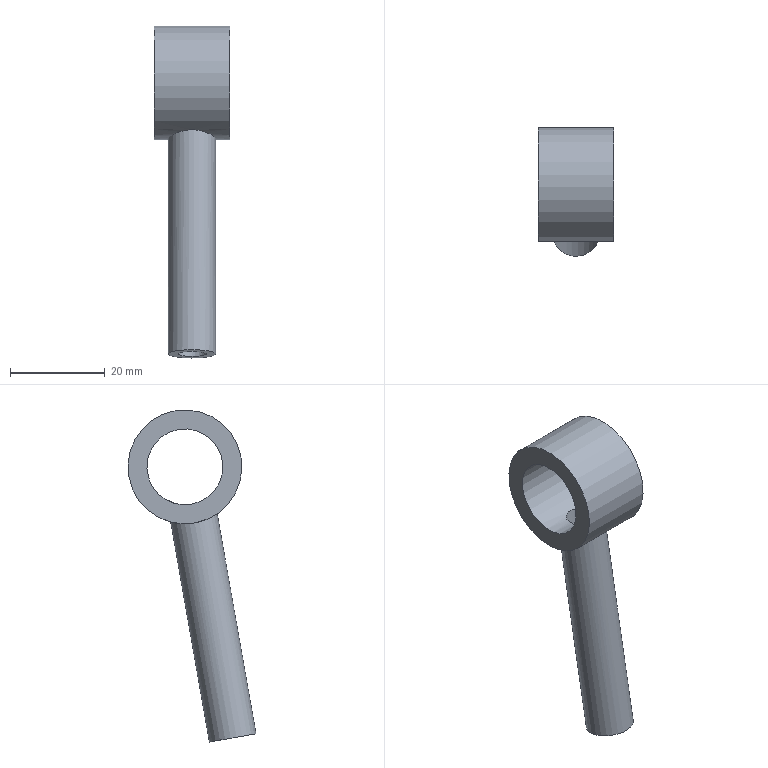Component | NX | SWING_ROD_2 | 1 solid | 7 faces | volume 6237 mm3 | cylinder 4 | plane 3 | commonest cylinder face diameters 24 x1 16 x1 10 x1 6 x1